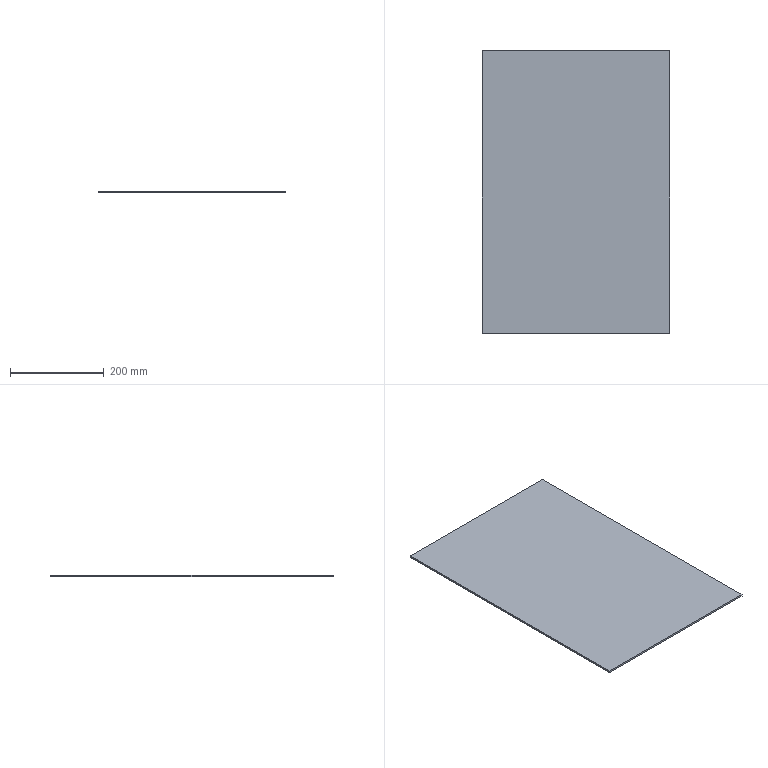Component | SolidWorks | w6-1 | 1 solid | 6 faces | box 400 x 602 x 4 mm | volume 963200 mm3 | plane 6
build123d program:
from build123d import *

# Parameters (mm, degrees)
SKETCH1_W           = 400
SKETCH1_H           = 602
BOSS_EXTRUDE1_DEPTH = 4


with BuildPart() as part:
    # Sketch1 → Boss-Extrude1 (new body)
    with BuildSketch(Plane.XY):
        Rectangle(SKETCH1_W, SKETCH1_H)
    extrude(amount=BOSS_EXTRUDE1_DEPTH)


solid = part.part

# Placed as in the assembly
solid = solid.moved(Location((0, 399.75, -7), (0, 0, 0)))
STEP:
#1=CARTESIAN_POINT('',(-7.874,27.589,-0.2756));
#2=VERTEX_POINT('',#1);
#3=CARTESIAN_POINT('',(-7.874,3.888,-0.2756));
#4=VERTEX_POINT('',#3);
#5=CARTESIAN_POINT('',(-7.874,3.888,-0.2756));
#6=DIRECTION('',(0.,-1.,0.));
#7=VECTOR('',#6,39.37);
#8=LINE('',#5,#7);
#9=EDGE_CURVE('',#2,#4,#8,.T.);
#10=ORIENTED_EDGE('',*,*,#9,.T.);
#11=CARTESIAN_POINT('',(-7.874,3.888,-0.1181));
#12=VERTEX_POINT('',#11);
#13=CARTESIAN_POINT('',(-7.874,3.888,-0.1181));
#14=DIRECTION('',(0.,0.,-1.));
#15=VECTOR('',#14,39.37);
#16=LINE('',#13,#15);
#17=EDGE_CURVE('',#12,#4,#16,.T.);
#18=ORIENTED_EDGE('',*,*,#17,.F.);
#19=CARTESIAN_POINT('',(-7.874,27.589,-0.1181));
#20=VERTEX_POINT('',#19);
#21=CARTESIAN_POINT('',(-7.874,3.888,-0.1181));
#22=DIRECTION('',(0.,-1.,0.));
#23=VECTOR('',#22,39.37);
#24=LINE('',#21,#23);
#25=EDGE_CURVE('',#20,#12,#24,.T.);
#26=ORIENTED_EDGE('',*,*,#25,.F.);
#27=CARTESIAN_POINT('',(-7.874,27.589,-0.1181));
#28=DIRECTION('',(0.,0.,-1.));
#29=VECTOR('',#28,39.37);
#30=LINE('',#27,#29);
#31=EDGE_CURVE('',#20,#2,#30,.T.);
#32=ORIENTED_EDGE('',*,*,#31,.T.);
#33=EDGE_LOOP('',(#10,#18,#26,#32));
#34=FACE_OUTER_BOUND('',#33,.T.);
#35=CARTESIAN_POINT('',(-7.874,3.888,-0.1181));
#36=DIRECTION('',(1.,0.,0.));
#37=DIRECTION('',(0.,0.,-1.));
#38=AXIS2_PLACEMENT_3D('',#35,#36,#37);
#39=PLANE('',#38);
#40=ADVANCED_FACE('',(#34),#39,.F.);
#41=CARTESIAN_POINT('',(7.874,3.888,-0.2756));
#42=VERTEX_POINT('',#41);
#43=CARTESIAN_POINT('',(7.874,3.888,-0.2756));
#44=DIRECTION('',(1.,0.,0.));
#45=VECTOR('',#44,39.37);
#46=LINE('',#43,#45);
#47=EDGE_CURVE('',#4,#42,#46,.T.);
#48=ORIENTED_EDGE('',*,*,#47,.T.);
#49=CARTESIAN_POINT('',(7.874,3.888,-0.1181));
#50=VERTEX_POINT('',#49);
#51=CARTESIAN_POINT('',(7.874,3.888,-0.1181));
#52=DIRECTION('',(0.,0.,-1.));
#53=VECTOR('',#52,39.37);
#54=LINE('',#51,#53);
#55=EDGE_CURVE('',#50,#42,#54,.T.);
#56=ORIENTED_EDGE('',*,*,#55,.F.);
#57=CARTESIAN_POINT('',(7.874,3.888,-0.1181));
#58=DIRECTION('',(1.,0.,0.));
#59=VECTOR('',#58,39.37);
#60=LINE('',#57,#59);
#61=EDGE_CURVE('',#12,#50,#60,.T.);
#62=ORIENTED_EDGE('',*,*,#61,.F.);
#63=ORIENTED_EDGE('',*,*,#17,.T.);
#64=EDGE_LOOP('',(#48,#56,#62,#63));
#65=FACE_OUTER_BOUND('',#64,.T.);
#66=CARTESIAN_POINT('',(7.874,3.888,-0.1181));
#67=DIRECTION('',(0.,1.,0.));
#68=DIRECTION('',(0.,0.,1.));
#69=AXIS2_PLACEMENT_3D('',#66,#67,#68);
#70=PLANE('',#69);
#71=ADVANCED_FACE('',(#65),#70,.F.);
#72=CARTESIAN_POINT('',(7.874,27.589,-0.2756));
#73=VERTEX_POINT('',#72);
#74=CARTESIAN_POINT('',(7.874,3.888,-0.2756));
#75=DIRECTION('',(0.,1.,0.));
#76=VECTOR('',#75,39.37);
#77=LINE('',#74,#76);
#78=EDGE_CURVE('',#42,#73,#77,.T.);
#79=ORIENTED_EDGE('',*,*,#78,.T.);
#80=CARTESIAN_POINT('',(7.874,27.589,-0.1181));
#81=VERTEX_POINT('',#80);
#82=CARTESIAN_POINT('',(7.874,27.589,-0.1181));
#83=DIRECTION('',(0.,0.,-1.));
#84=VECTOR('',#83,39.37);
#85=LINE('',#82,#84);
#86=EDGE_CURVE('',#81,#73,#85,.T.);
#87=ORIENTED_EDGE('',*,*,#86,.F.);
#88=CARTESIAN_POINT('',(7.874,3.888,-0.1181));
#89=DIRECTION('',(0.,1.,0.));
#90=VECTOR('',#89,39.37);
#91=LINE('',#88,#90);
#92=EDGE_CURVE('',#50,#81,#91,.T.);
#93=ORIENTED_EDGE('',*,*,#92,.F.);
#94=ORIENTED_EDGE('',*,*,#55,.T.);
#95=EDGE_LOOP('',(#79,#87,#93,#94));
#96=FACE_OUTER_BOUND('',#95,.T.);
#97=CARTESIAN_POINT('',(7.874,3.888,-0.1181));
#98=DIRECTION('',(-1.,0.,0.));
#99=DIRECTION('',(0.,0.,1.));
#100=AXIS2_PLACEMENT_3D('',#97,#98,#99);
#101=PLANE('',#100);
#102=ADVANCED_FACE('',(#96),#101,.F.);
#103=CARTESIAN_POINT('',(7.874,27.589,-0.2756));
#104=DIRECTION('',(-1.,0.,0.));
#105=VECTOR('',#104,39.37);
#106=LINE('',#103,#105);
#107=EDGE_CURVE('',#73,#2,#106,.T.);
#108=ORIENTED_EDGE('',*,*,#107,.T.);
#109=ORIENTED_EDGE('',*,*,#31,.F.);
#110=CARTESIAN_POINT('',(7.874,27.589,-0.1181));
#111=DIRECTION('',(-1.,0.,0.));
#112=VECTOR('',#111,39.37);
#113=LINE('',#110,#112);
#114=EDGE_CURVE('',#81,#20,#113,.T.);
#115=ORIENTED_EDGE('',*,*,#114,.F.);
#116=ORIENTED_EDGE('',*,*,#86,.T.);
#117=EDGE_LOOP('',(#108,#109,#115,#116));
#118=FACE_OUTER_BOUND('',#117,.T.);
#119=CARTESIAN_POINT('',(7.874,27.589,-0.1181));
#120=DIRECTION('',(0.,-1.,0.));
#121=DIRECTION('',(0.,0.,-1.));
#122=AXIS2_PLACEMENT_3D('',#119,#120,#121);
#123=PLANE('',#122);
#124=ADVANCED_FACE('',(#118),#123,.F.);
#125=ORIENTED_EDGE('',*,*,#25,.T.);
#126=ORIENTED_EDGE('',*,*,#61,.T.);
#127=ORIENTED_EDGE('',*,*,#92,.T.);
#128=ORIENTED_EDGE('',*,*,#114,.T.);
#129=EDGE_LOOP('',(#125,#126,#127,#128));
#130=FACE_OUTER_BOUND('',#129,.T.);
#131=CARTESIAN_POINT('',(0.,15.738,-0.1181));
#132=DIRECTION('',(0.,0.,1.));
#133=DIRECTION('',(1.,0.,0.));
#134=AXIS2_PLACEMENT_3D('',#131,#132,#133);
#135=PLANE('',#134);
#136=ADVANCED_FACE('',(#130),#135,.T.);
#137=ORIENTED_EDGE('',*,*,#9,.F.);
#138=ORIENTED_EDGE('',*,*,#107,.F.);
#139=ORIENTED_EDGE('',*,*,#78,.F.);
#140=ORIENTED_EDGE('',*,*,#47,.F.);
#141=EDGE_LOOP('',(#137,#138,#139,#140));
#142=FACE_OUTER_BOUND('',#141,.T.);
#143=CARTESIAN_POINT('',(0.,15.738,-0.2756));
#144=DIRECTION('',(0.,0.,1.));
#145=DIRECTION('',(1.,0.,0.));
#146=AXIS2_PLACEMENT_3D('',#143,#144,#145);
#147=PLANE('',#146);
#148=ADVANCED_FACE('',(#142),#147,.F.);
#149=CLOSED_SHELL('',(#40,#71,#102,#124,#136,#148));
#150=MANIFOLD_SOLID_BREP('',#149);
#151=CARTESIAN_POINT('',(0.,0.,0.));
#152=DIRECTION('',(0.,0.,1.));
#153=DIRECTION('',(1.,0.,0.));
#154=AXIS2_PLACEMENT_3D('',#151,#152,#153);
#155=(LENGTH_UNIT()NAMED_UNIT(*)SI_UNIT($,.METRE.));
#156=LENGTH_MEASURE_WITH_UNIT(LENGTH_MEASURE(0.0254),#155);
#157=DIMENSIONAL_EXPONENTS(1.,0.,0.,0.,0.,0.,0.);
#158=(CONVERSION_BASED_UNIT('',#156)LENGTH_UNIT()NAMED_UNIT(#157));
#159=UNCERTAINTY_MEASURE_WITH_UNIT(LENGTH_MEASURE(0.00001),#158,'','');
#160=(NAMED_UNIT(*)PLANE_ANGLE_UNIT()SI_UNIT($,.RADIAN.));
#161=(NAMED_UNIT(*)SI_UNIT($,.STERADIAN.)SOLID_ANGLE_UNIT());
#162=(GEOMETRIC_REPRESENTATION_CONTEXT(3)GLOBAL_UNCERTAINTY_ASSIGNED_CONTEXT((#159))GLOBAL_UNIT_ASSIGNED_CONTEXT((#158,#160,#161))REPRESENTATION_CONTEXT('',''));
#163=ADVANCED_BREP_SHAPE_REPRESENTATION('',(#150,#154),#162);
#164=COLOUR_RGB('',0.7922,0.8196,0.9333);
#165=FILL_AREA_STYLE_COLOUR('',#164);
#166=FILL_AREA_STYLE('',(#165));
#167=SURFACE_STYLE_FILL_AREA(#166);
#168=SURFACE_SIDE_STYLE('',(#167));
#169=SURFACE_STYLE_USAGE(.BOTH.,#168);
#170=PRESENTATION_STYLE_ASSIGNMENT((#169));
#171=STYLED_ITEM('',(#170),#150);
#172=PRESENTATION_LAYER_ASSIGNMENT('','',(#171));
#173=(LENGTH_UNIT()NAMED_UNIT(*)SI_UNIT($,.METRE.));
#174=LENGTH_MEASURE_WITH_UNIT(LENGTH_MEASURE(0.0254),#173);
#175=DIMENSIONAL_EXPONENTS(1.,0.,0.,0.,0.,0.,0.);
#176=(CONVERSION_BASED_UNIT('',#174)LENGTH_UNIT()NAMED_UNIT(#175));
#177=UNCERTAINTY_MEASURE_WITH_UNIT(LENGTH_MEASURE(0.00001),#176,'','');
#178=(NAMED_UNIT(*)PLANE_ANGLE_UNIT()SI_UNIT($,.RADIAN.));
#179=(NAMED_UNIT(*)SI_UNIT($,.STERADIAN.)SOLID_ANGLE_UNIT());
#180=(GEOMETRIC_REPRESENTATION_CONTEXT(3)GLOBAL_UNCERTAINTY_ASSIGNED_CONTEXT((#177))GLOBAL_UNIT_ASSIGNED_CONTEXT((#176,#178,#179))REPRESENTATION_CONTEXT('',''));
#181=MECHANICAL_DESIGN_GEOMETRIC_PRESENTATION_REPRESENTATION('',(#171),#180);